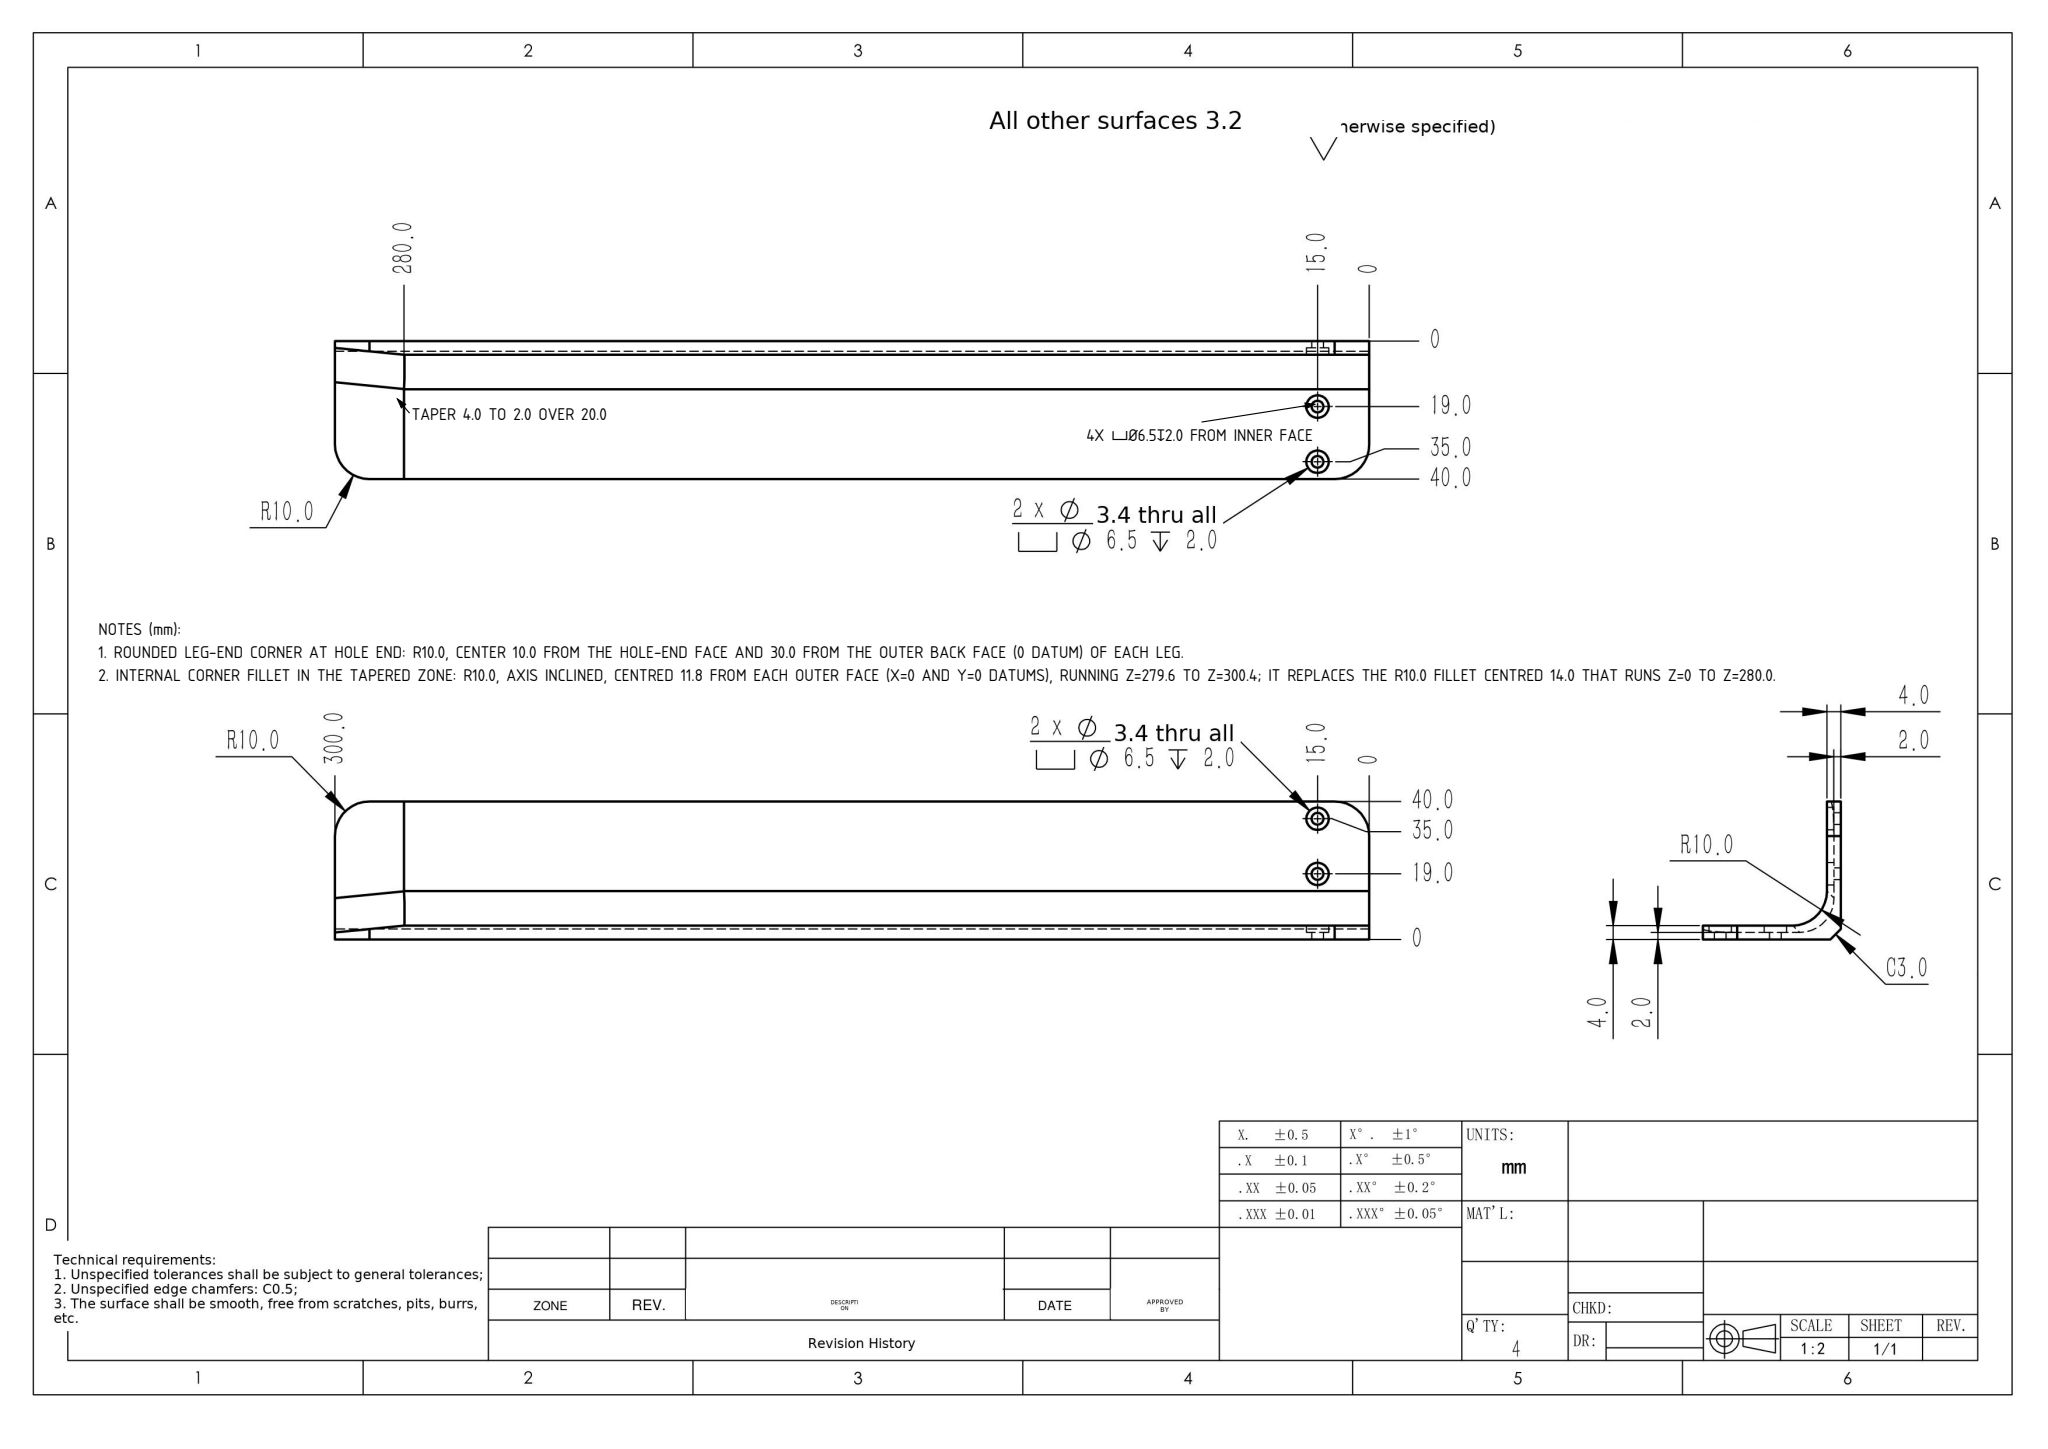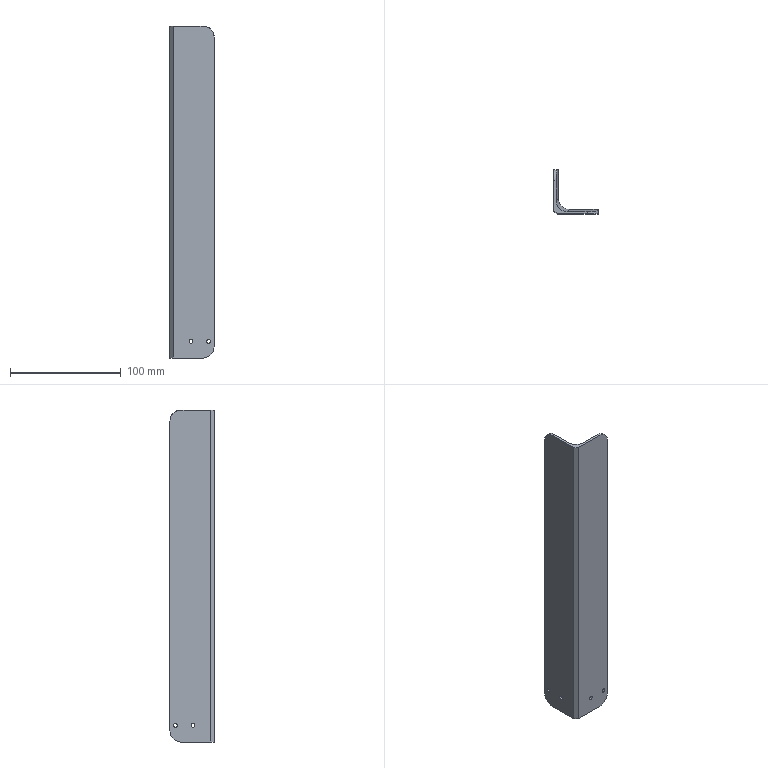Part | SolidWorks | mm | 1 solid | 37 faces | box 40 x 40 x 300 mm | volume 94211 mm3 | cylinder 22 | plane 15 | commonest cylinder face diameters 6.5 x8 3.4 x8 20 x6
Drawing notes:
ROUNDED LEG-END CORNER AT HOLE END: R10.0, CENTER 10.0 FROM THE HOLE-END FACE AND 30.0 FROM THE OUTER BACK FACE (0 DATUM) OF EACH LEG. | from the solid: cylinders [20.0,'x',[null,30.0,10.0],4.0] and [20.0,'y',[30.0,null,10.0],4.0]
WALL TRANSITION IS A TAPER, NOT A STEP: INNER WALL FACE RUNS AT 5.7 DEG TO THE Z AXIS OVER THE 20.0 LENGTH FROM Z=280.0 TO Z=300.0 (Z=0 = HOLE END FACE), TAKING WALL FROM 4.0 THICK (INNER FACE AT X=4.0 / Y=4.0) TO 2.0 THICK (INNER FACE AT X=2.0 / Y=2.0) AT Z=300.0. | from the solid: inclined_planes 5.7 deg, bbox_from [2.0,12.0,280.0] size [2.0,28.0,20.0] and [12.0,2.0,280.0] size [28.0,2.0,20.0]; axis_planes x=4.0 and y=4.0 extend z 0-280.0
INTERNAL CORNER FILLET IN THE TAPERED ZONE: R10.0, AXIS INCLINED, CENTRED 11.8 FROM EACH OUTER FACE (X=0 AND Y=0 DATUMS), RUNNING Z=279.6 TO Z=300.4; IT REPLACES THE R10.0 FILLET CENTRED 14.0 THAT RUNS Z=0 TO Z=280.0. | from the solid: cylinders: concave arc dia 20.0 inclined at (11.8,11.8) from 279.6 to 300.4, 89 deg; concave arc dia 20.0 axis z at (14.0,14.0) from 0.0 to 280.0
COUNTERBORE DIRECTION: 4X Ø3.4 THRU DRILLED FROM THE OUTER BACK FACE (X=0 / Y=0 DATUM), Ø6.5 CBORE 2.0 DEEP MACHINED FROM THE INNER FACE (X=4.0 / Y=4.0), I.E. CBORE SPANS 2.0 TO 4.0 FROM THE DATUM FACE; HOLE AXES AT Z=15.0, AT 19.0 AND 35.0 FROM THE OPPOSITE OUTER FACE. | from the solid: cylinders: hole 3.4 axis x/y at (19.0/35.0, z=15.0) from 0.0 to 2.0; hole 6.5 same axes from 2.0 to 4.0